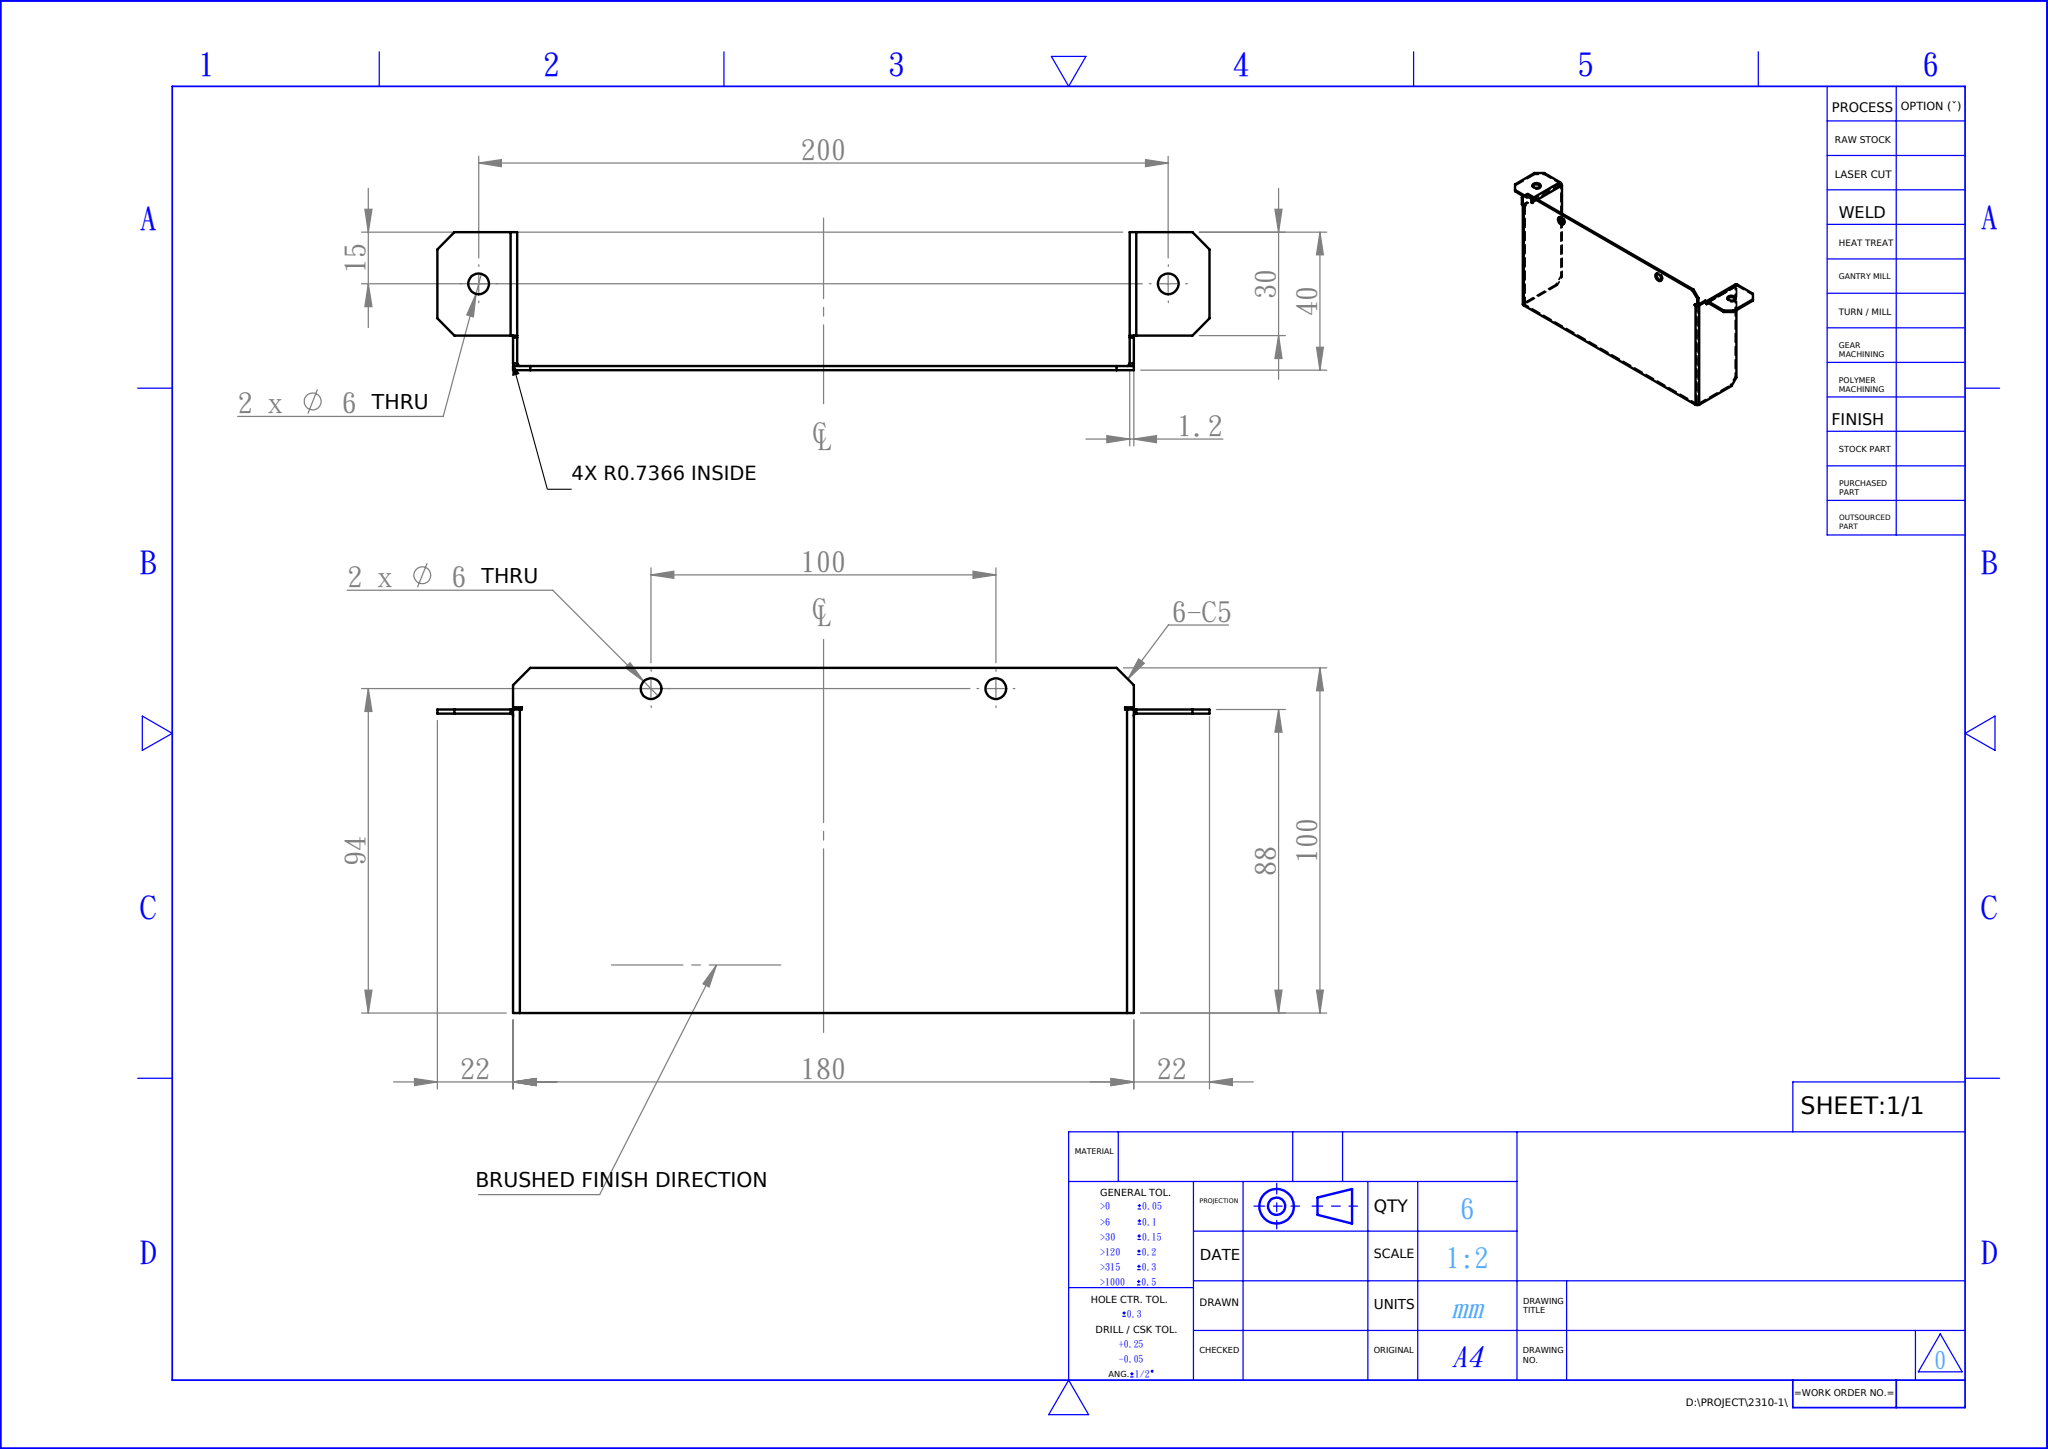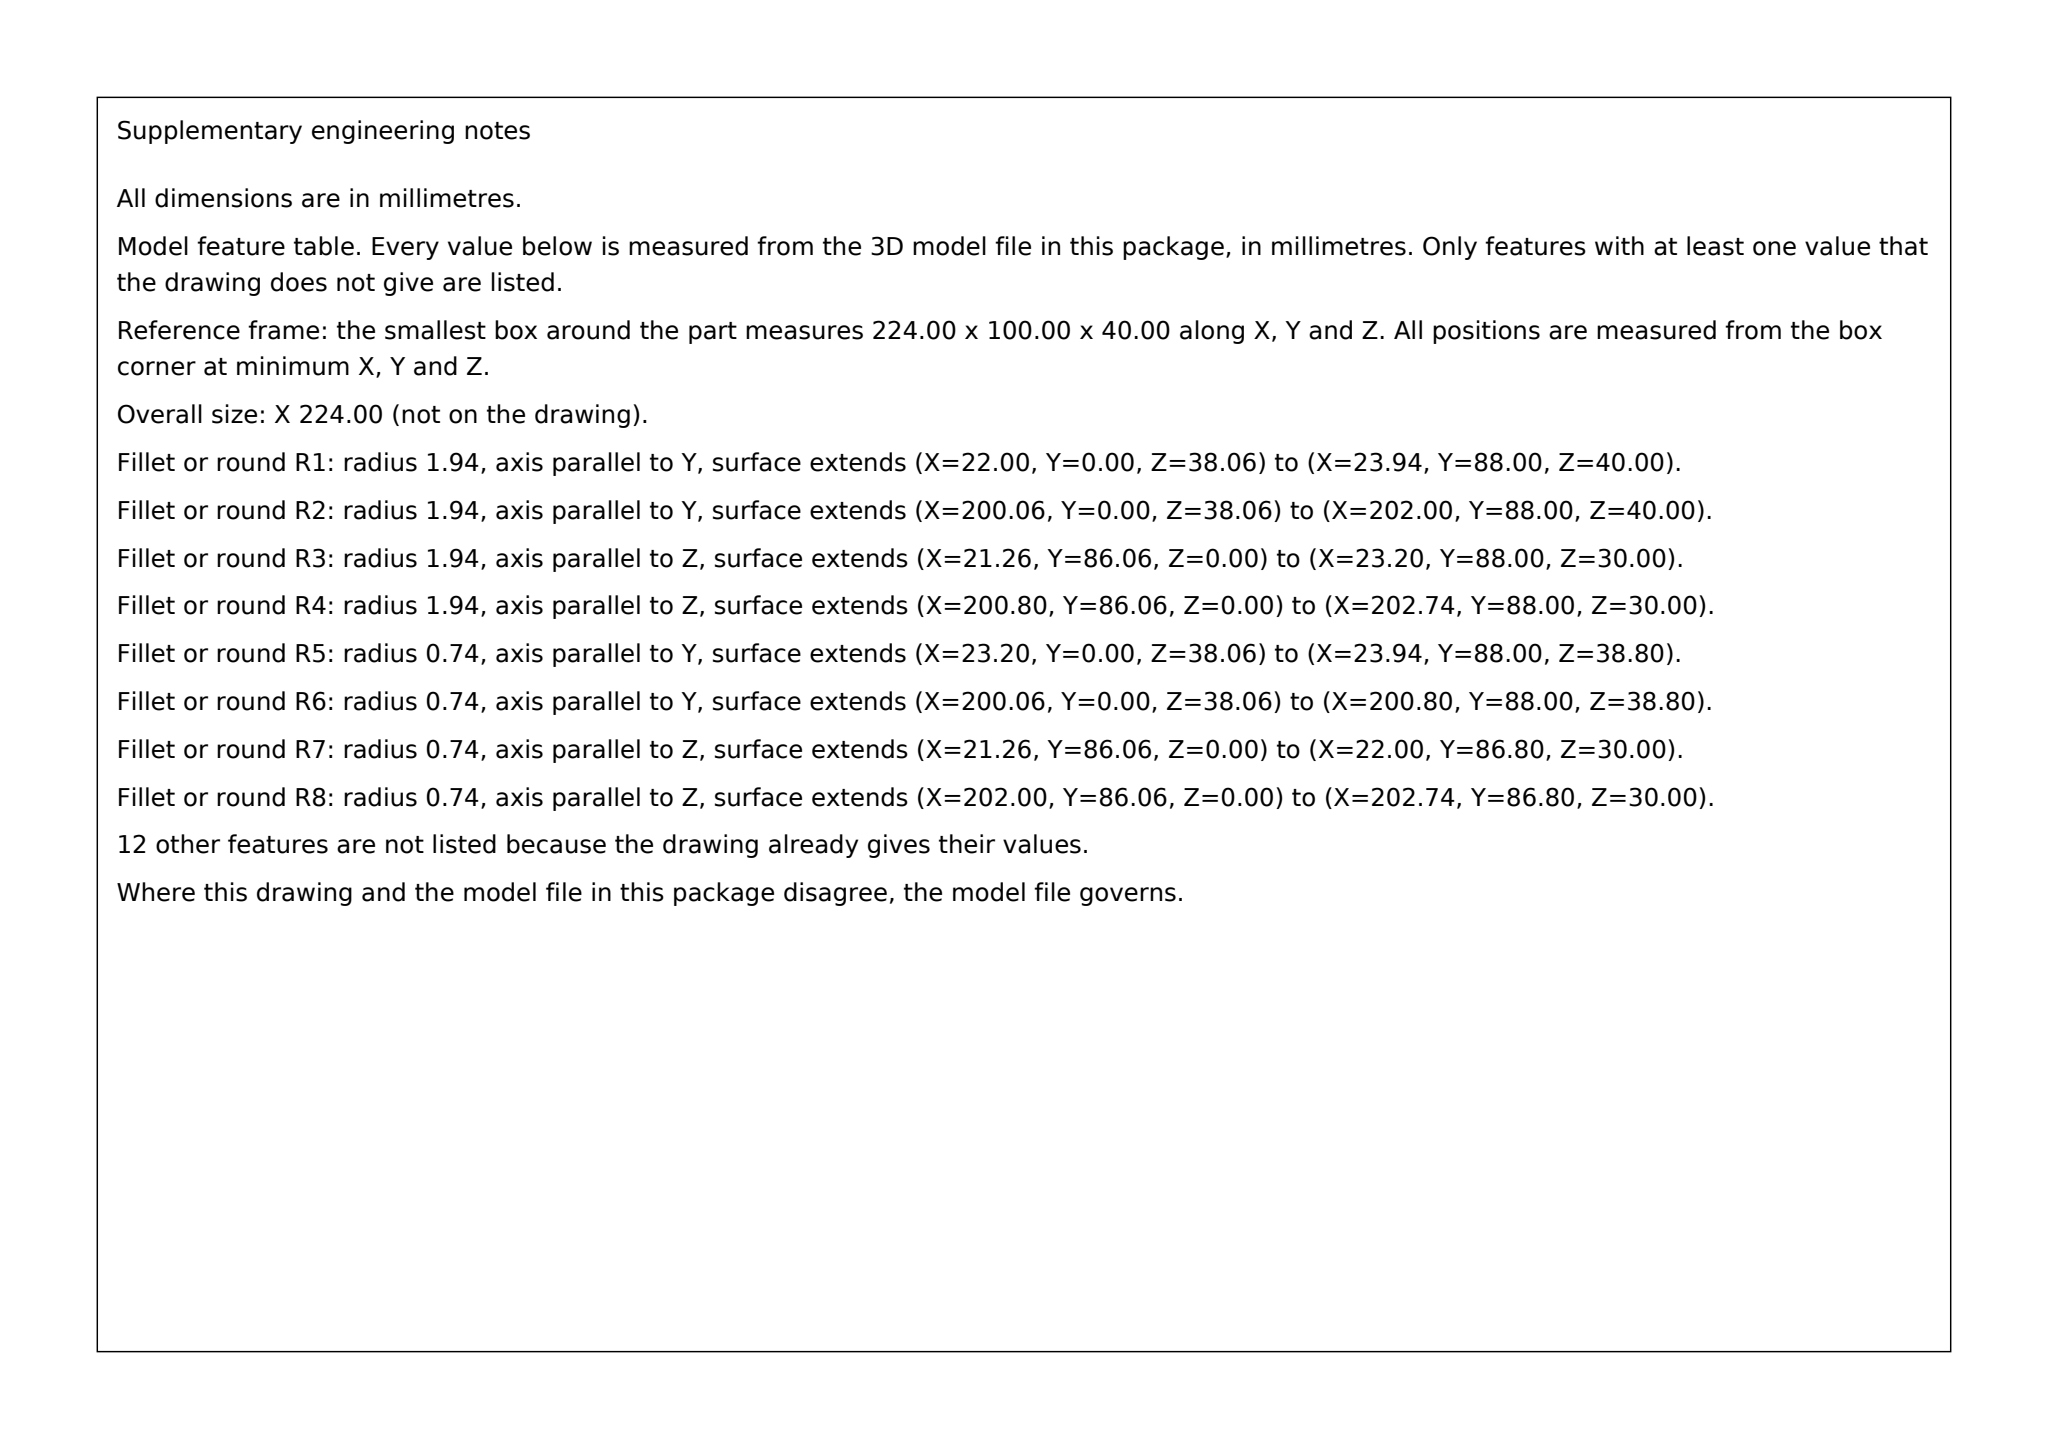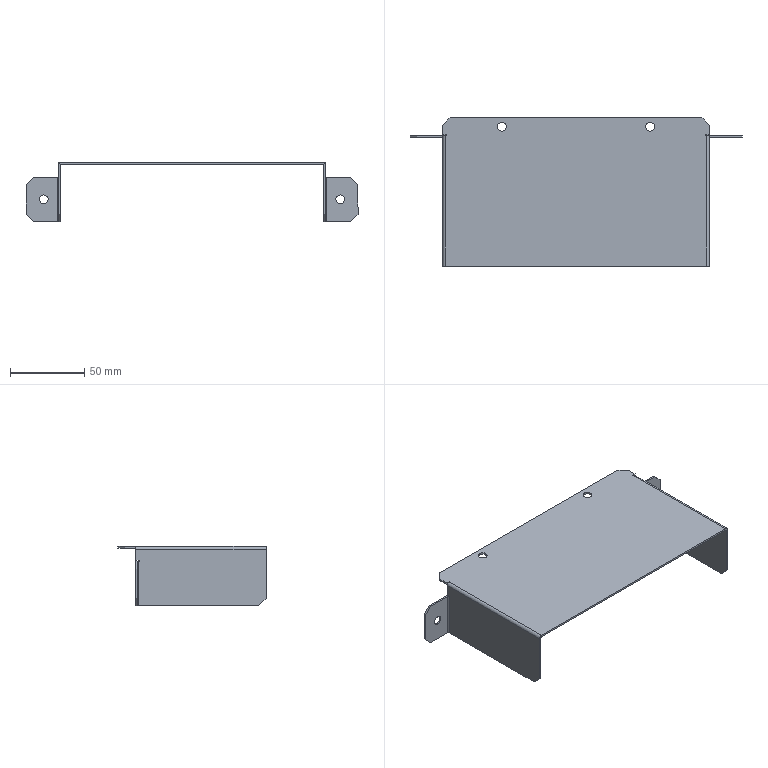Part | SolidWorks | mm | 1 solid | 70 faces | box 224 x 100 x 40 mm | volume 30953 mm3 | plane 54 | cylinder 16 | commonest cylinder face diameters 6 x8 3.873 x4 1.473 x4